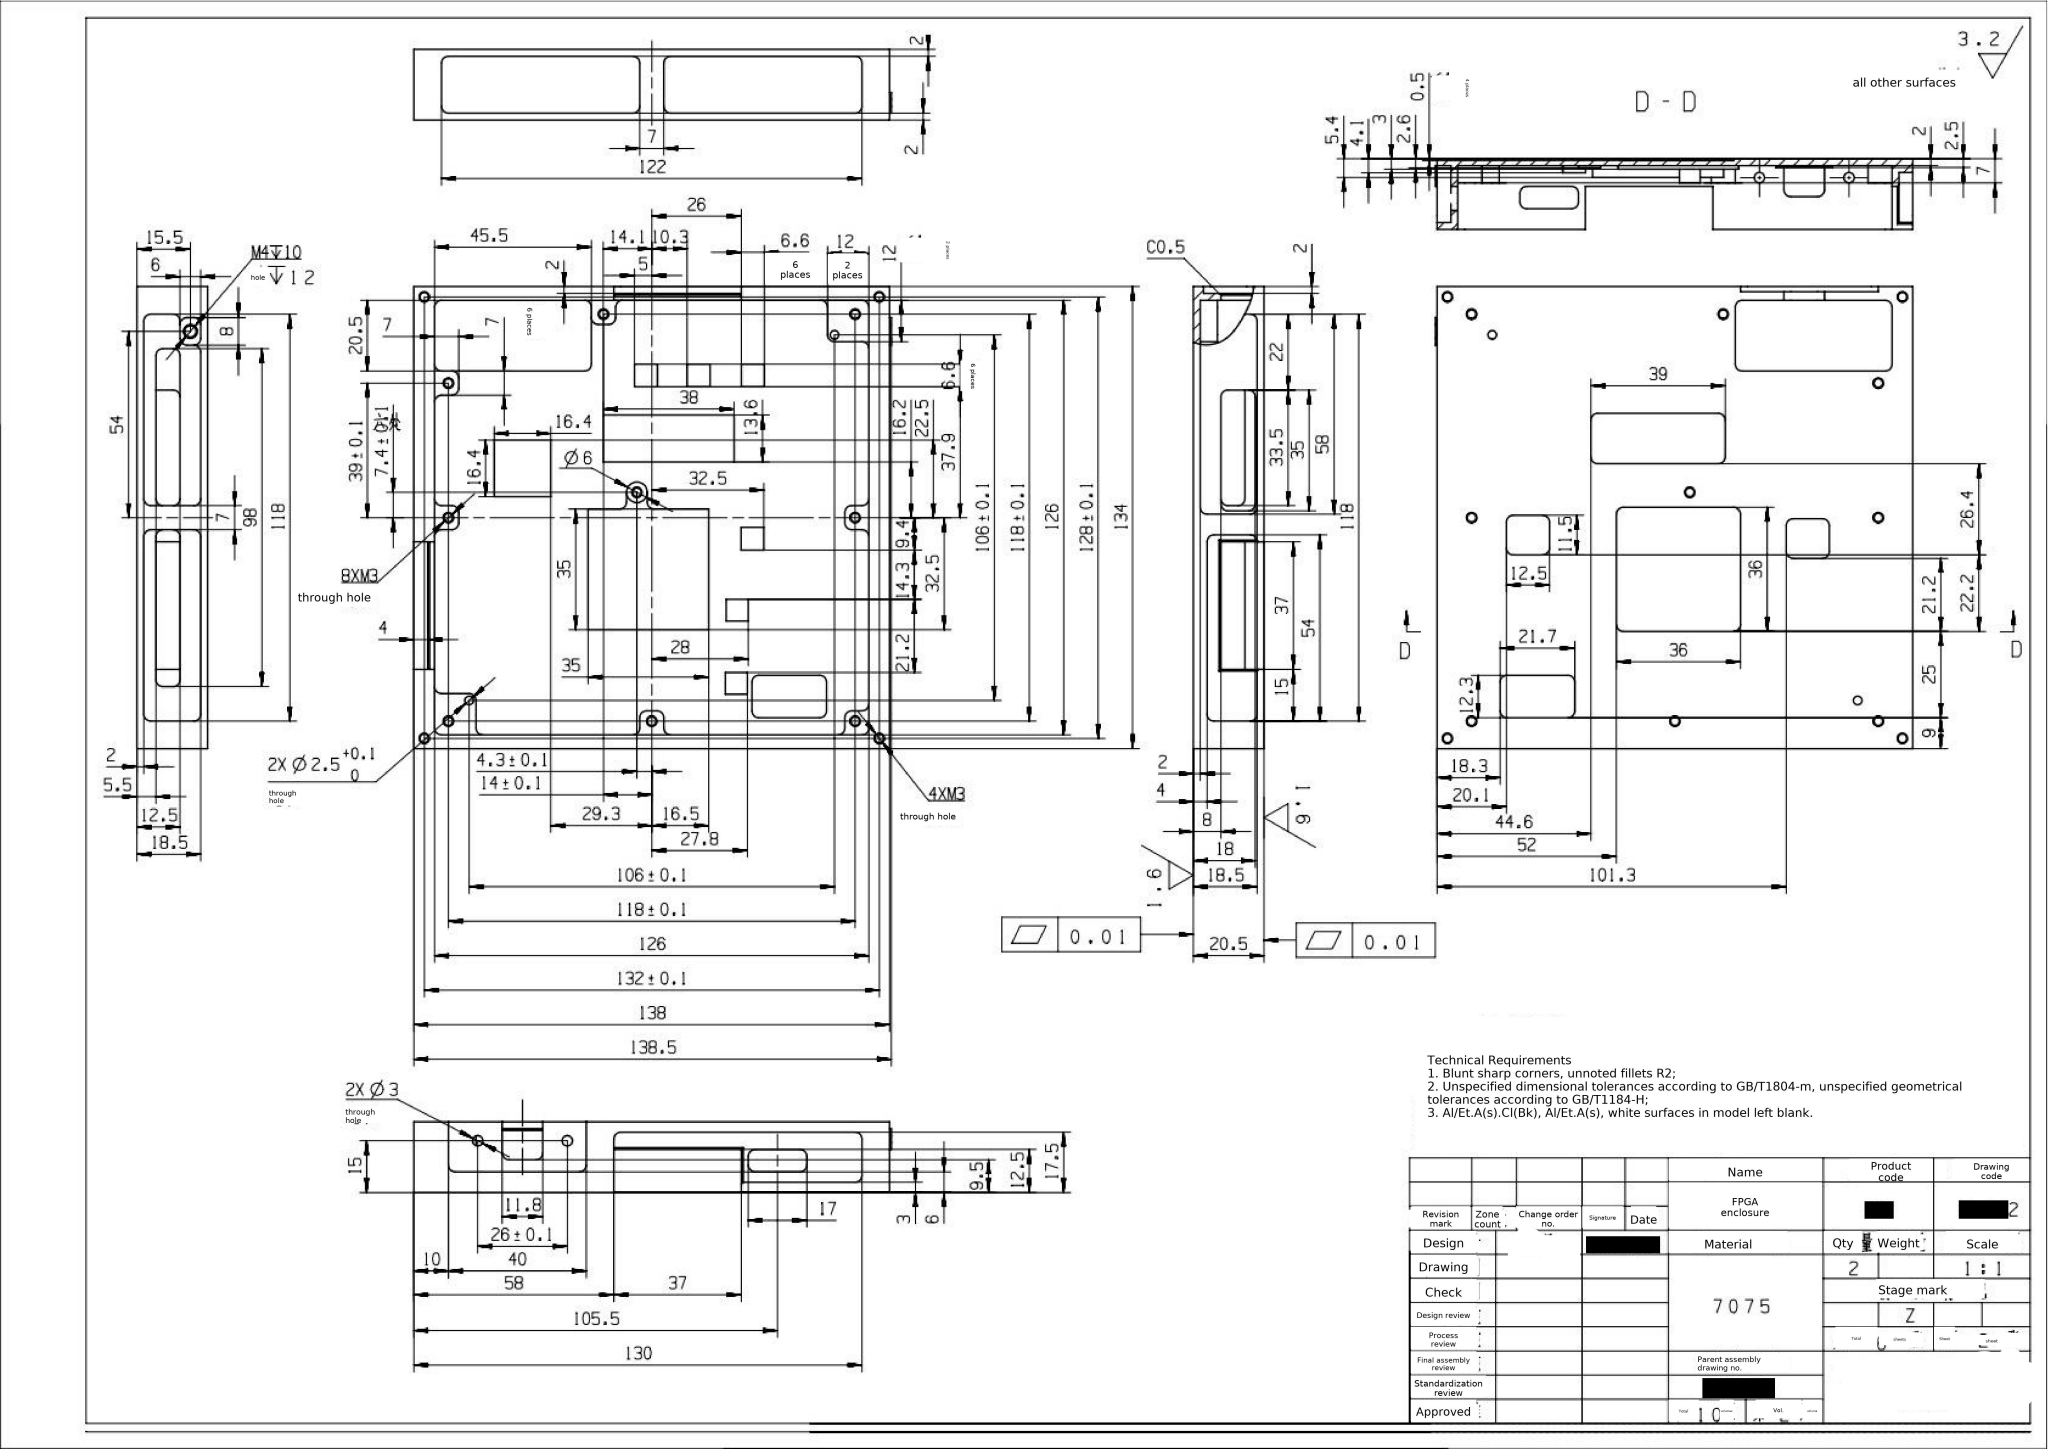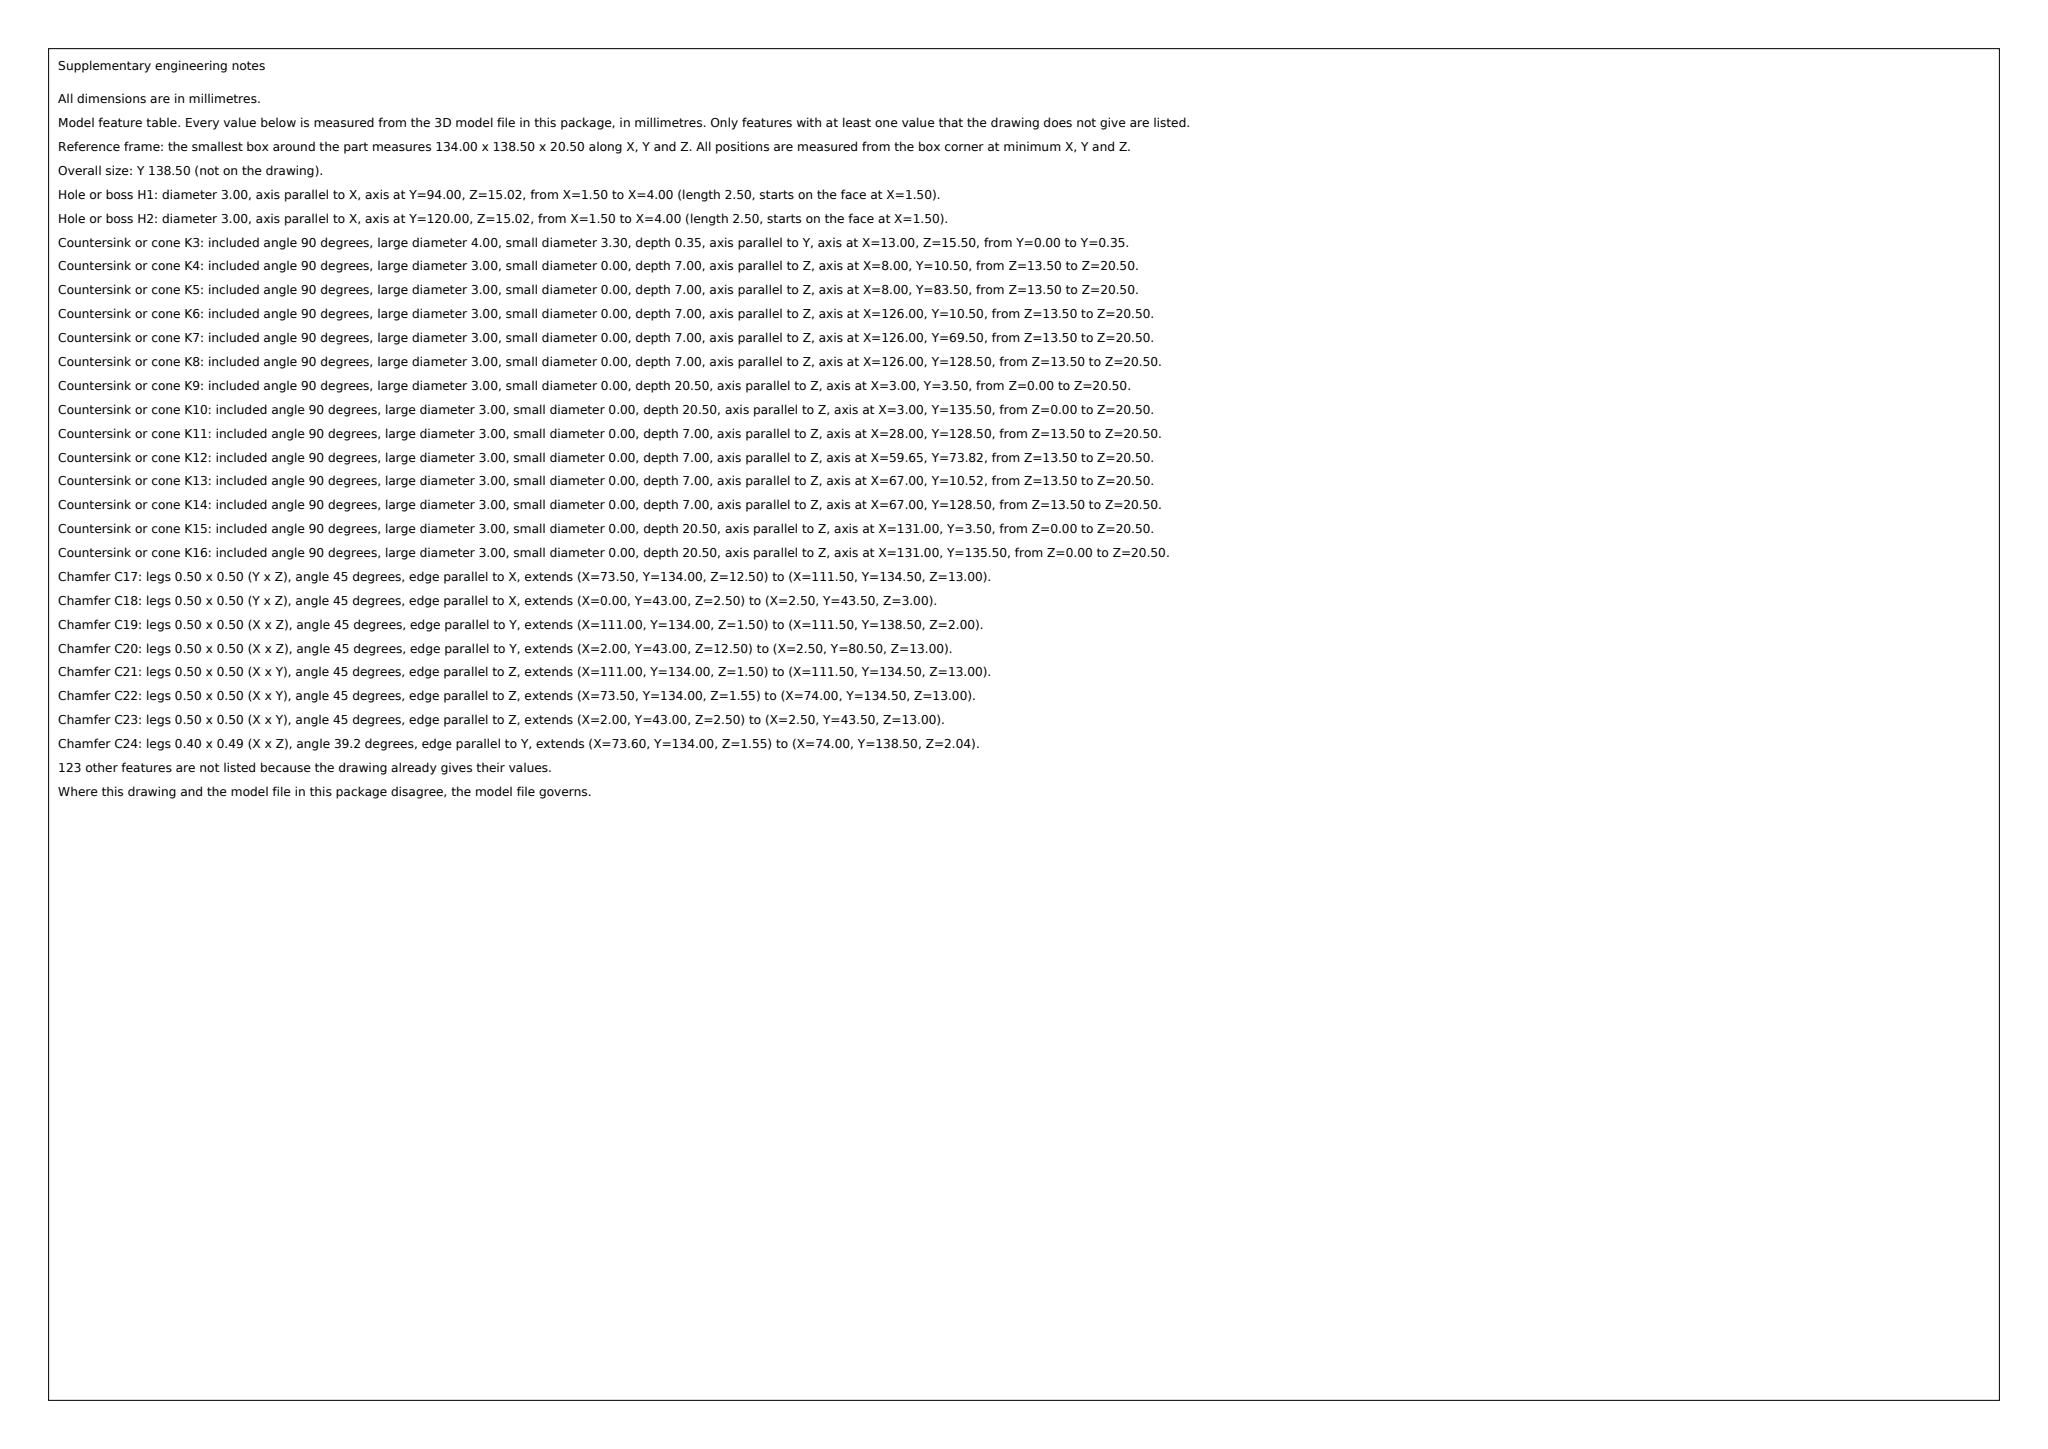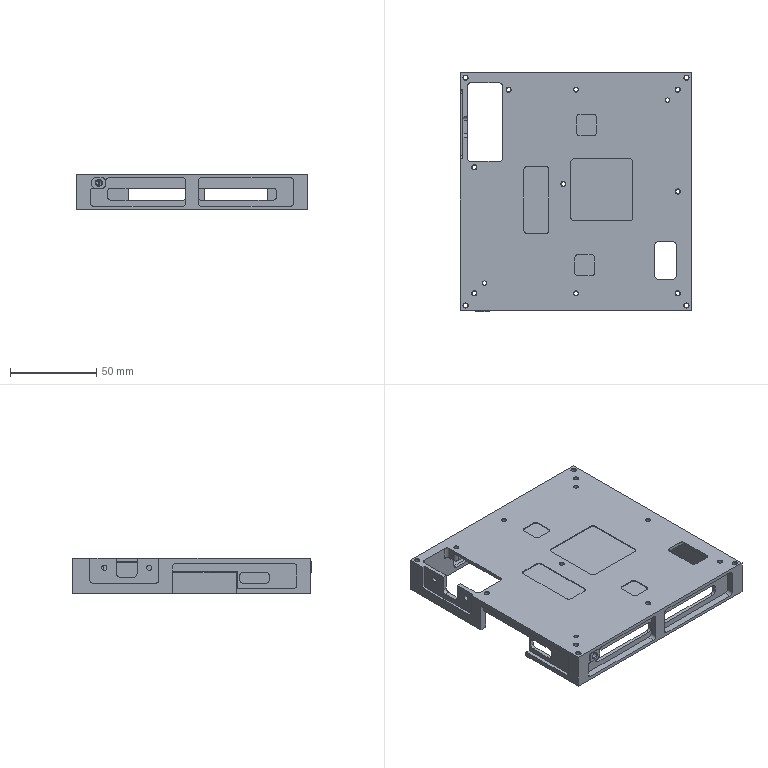Part | SolidWorks | mm | material 7075 | 1 solid | 390 faces | box 134 x 138.5 x 20.5 mm | volume 62053 mm3 | plane 188 | cylinder 146 | cone 56 | commonest cylinder face diameters 4 x108 2.5 x30 3 x4 3.3 x2 6 x2